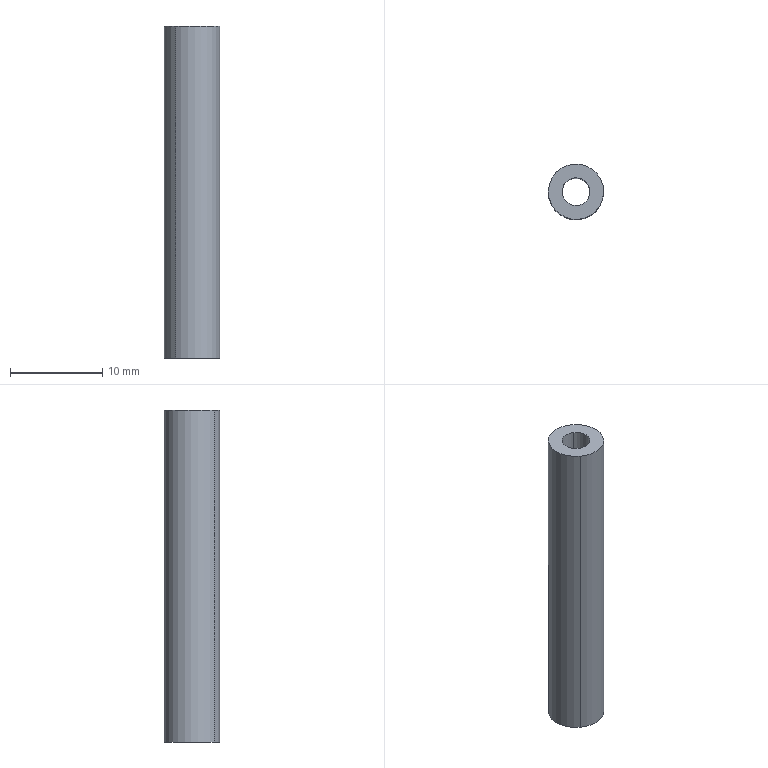Component | SolidWorks | UpperAndLowerPlateSupportColumn-3 | 1 solid | 6 faces | box 6 x 6 x 36 mm | volume 763 mm3 | cylinder 4 | plane 2 | commonest cylinder face diameters 3 x2 6 x2
build123d program:
from build123d import *

# Parameters (mm, degrees)
SKETCH1_R           = 3
SKETCH1_R_2         = 1.5
BOSS_EXTRUDE1_DEPTH = 36


with BuildPart() as part:
    # Sketch1 → Boss-Extrude1 (new body)
    with BuildSketch(Plane.XY):
        Circle(SKETCH1_R)
        Circle(SKETCH1_R_2, mode=Mode.SUBTRACT)
    extrude(amount=BOSS_EXTRUDE1_DEPTH)


solid = part.part

# Placed as in the assembly
solid = solid.moved(Location((14.261, -183.575, 1001.6), (0, 0, 0)))
STEP:
#1=CARTESIAN_POINT('',(0.5265,-7.275,40.85));
#2=VERTEX_POINT('',#1);
#3=CARTESIAN_POINT('',(0.5964,-7.18,40.85));
#4=VERTEX_POINT('',#3);
#5=CARTESIAN_POINT('',(0.5615,-7.227,40.85));
#6=DIRECTION('',(0.,0.,1.));
#7=DIRECTION('',(0.5916,0.8062,0.));
#8=AXIS2_PLACEMENT_3D('',#5,#6,#7);
#9=CIRCLE('',#8,0.05906);
#10=EDGE_CURVE('',#2,#4,#9,.T.);
#11=ORIENTED_EDGE('',*,*,#10,.T.);
#12=CARTESIAN_POINT('',(0.5964,-7.18,39.433));
#13=VERTEX_POINT('',#12);
#14=CARTESIAN_POINT('',(0.5964,-7.18,40.85));
#15=DIRECTION('',(0.,0.,-1.));
#16=VECTOR('',#15,39.37);
#17=LINE('',#14,#16);
#18=EDGE_CURVE('',#4,#13,#17,.T.);
#19=ORIENTED_EDGE('',*,*,#18,.T.);
#20=CARTESIAN_POINT('',(0.5265,-7.275,39.433));
#21=VERTEX_POINT('',#20);
#22=CARTESIAN_POINT('',(0.5615,-7.227,39.433));
#23=DIRECTION('',(0.,0.,1.));
#24=DIRECTION('',(0.5916,0.8062,0.));
#25=AXIS2_PLACEMENT_3D('',#22,#23,#24);
#26=CIRCLE('',#25,0.05906);
#27=EDGE_CURVE('',#21,#13,#26,.T.);
#28=ORIENTED_EDGE('',*,*,#27,.F.);
#29=CARTESIAN_POINT('',(0.5265,-7.275,40.85));
#30=DIRECTION('',(0.,0.,-1.));
#31=VECTOR('',#30,39.37);
#32=LINE('',#29,#31);
#33=EDGE_CURVE('',#2,#21,#32,.T.);
#34=ORIENTED_EDGE('',*,*,#33,.F.);
#35=EDGE_LOOP('',(#11,#19,#28,#34));
#36=FACE_OUTER_BOUND('',#35,.T.);
#37=CARTESIAN_POINT('',(0.5615,-7.227,40.85));
#38=DIRECTION('',(0.,0.,-1.));
#39=DIRECTION('',(-0.5916,-0.8062,0.));
#40=AXIS2_PLACEMENT_3D('',#37,#38,#39);
#41=CYLINDRICAL_SURFACE('',#40,0.05906);
#42=ADVANCED_FACE('',(#36),#41,.F.);
#43=CARTESIAN_POINT('',(0.6313,-7.132,40.85));
#44=VERTEX_POINT('',#43);
#45=CARTESIAN_POINT('',(0.4916,-7.323,40.85));
#46=VERTEX_POINT('',#45);
#47=CARTESIAN_POINT('',(0.5615,-7.227,40.85));
#48=DIRECTION('',(0.,0.,1.));
#49=DIRECTION('',(0.5916,0.8062,0.));
#50=AXIS2_PLACEMENT_3D('',#47,#48,#49);
#51=CIRCLE('',#50,0.1181);
#52=EDGE_CURVE('',#44,#46,#51,.T.);
#53=ORIENTED_EDGE('',*,*,#52,.F.);
#54=CARTESIAN_POINT('',(0.6313,-7.132,39.433));
#55=VERTEX_POINT('',#54);
#56=CARTESIAN_POINT('',(0.6313,-7.132,40.85));
#57=DIRECTION('',(0.,0.,-1.));
#58=VECTOR('',#57,39.37);
#59=LINE('',#56,#58);
#60=EDGE_CURVE('',#44,#55,#59,.T.);
#61=ORIENTED_EDGE('',*,*,#60,.T.);
#62=CARTESIAN_POINT('',(0.4916,-7.323,39.433));
#63=VERTEX_POINT('',#62);
#64=CARTESIAN_POINT('',(0.5615,-7.227,39.433));
#65=DIRECTION('',(0.,0.,1.));
#66=DIRECTION('',(0.5916,0.8062,0.));
#67=AXIS2_PLACEMENT_3D('',#64,#65,#66);
#68=CIRCLE('',#67,0.1181);
#69=EDGE_CURVE('',#55,#63,#68,.T.);
#70=ORIENTED_EDGE('',*,*,#69,.T.);
#71=CARTESIAN_POINT('',(0.4916,-7.323,40.85));
#72=DIRECTION('',(0.,0.,-1.));
#73=VECTOR('',#72,39.37);
#74=LINE('',#71,#73);
#75=EDGE_CURVE('',#46,#63,#74,.T.);
#76=ORIENTED_EDGE('',*,*,#75,.F.);
#77=EDGE_LOOP('',(#53,#61,#70,#76));
#78=FACE_OUTER_BOUND('',#77,.T.);
#79=CARTESIAN_POINT('',(0.5615,-7.227,40.85));
#80=DIRECTION('',(0.,0.,-1.));
#81=DIRECTION('',(-0.5916,-0.8062,0.));
#82=AXIS2_PLACEMENT_3D('',#79,#80,#81);
#83=CYLINDRICAL_SURFACE('',#82,0.1181);
#84=ADVANCED_FACE('',(#78),#83,.T.);
#85=CARTESIAN_POINT('',(0.5615,-7.227,40.85));
#86=DIRECTION('',(0.,0.,1.));
#87=DIRECTION('',(0.5916,0.8062,0.));
#88=AXIS2_PLACEMENT_3D('',#85,#86,#87);
#89=CIRCLE('',#88,0.1181);
#90=EDGE_CURVE('',#46,#44,#89,.T.);
#91=ORIENTED_EDGE('',*,*,#90,.T.);
#92=ORIENTED_EDGE('',*,*,#52,.T.);
#93=EDGE_LOOP('',(#91,#92));
#94=FACE_OUTER_BOUND('',#93,.T.);
#95=ORIENTED_EDGE('',*,*,#10,.F.);
#96=CARTESIAN_POINT('',(0.5615,-7.227,40.85));
#97=DIRECTION('',(0.,0.,1.));
#98=DIRECTION('',(0.5916,0.8062,0.));
#99=AXIS2_PLACEMENT_3D('',#96,#97,#98);
#100=CIRCLE('',#99,0.05906);
#101=EDGE_CURVE('',#4,#2,#100,.T.);
#102=ORIENTED_EDGE('',*,*,#101,.F.);
#103=EDGE_LOOP('',(#95,#102));
#104=FACE_BOUND('',#103,.T.);
#105=CARTESIAN_POINT('',(0.5615,-7.227,40.85));
#106=DIRECTION('',(0.,0.,1.));
#107=DIRECTION('',(0.5916,0.8062,0.));
#108=AXIS2_PLACEMENT_3D('',#105,#106,#107);
#109=PLANE('',#108);
#110=ADVANCED_FACE('',(#94,#104),#109,.T.);
#111=CARTESIAN_POINT('',(0.5615,-7.227,39.433));
#112=DIRECTION('',(0.,0.,1.));
#113=DIRECTION('',(0.5916,0.8062,0.));
#114=AXIS2_PLACEMENT_3D('',#111,#112,#113);
#115=CIRCLE('',#114,0.1181);
#116=EDGE_CURVE('',#63,#55,#115,.T.);
#117=ORIENTED_EDGE('',*,*,#116,.F.);
#118=ORIENTED_EDGE('',*,*,#69,.F.);
#119=EDGE_LOOP('',(#117,#118));
#120=FACE_OUTER_BOUND('',#119,.T.);
#121=ORIENTED_EDGE('',*,*,#27,.T.);
#122=CARTESIAN_POINT('',(0.5615,-7.227,39.433));
#123=DIRECTION('',(0.,0.,1.));
#124=DIRECTION('',(0.5916,0.8062,0.));
#125=AXIS2_PLACEMENT_3D('',#122,#123,#124);
#126=CIRCLE('',#125,0.05906);
#127=EDGE_CURVE('',#13,#21,#126,.T.);
#128=ORIENTED_EDGE('',*,*,#127,.T.);
#129=EDGE_LOOP('',(#121,#128));
#130=FACE_BOUND('',#129,.T.);
#131=CARTESIAN_POINT('',(0.5615,-7.227,39.433));
#132=DIRECTION('',(0.,0.,1.));
#133=DIRECTION('',(0.5916,0.8062,0.));
#134=AXIS2_PLACEMENT_3D('',#131,#132,#133);
#135=PLANE('',#134);
#136=ADVANCED_FACE('',(#120,#130),#135,.F.);
#137=ORIENTED_EDGE('',*,*,#60,.F.);
#138=ORIENTED_EDGE('',*,*,#90,.F.);
#139=ORIENTED_EDGE('',*,*,#75,.T.);
#140=ORIENTED_EDGE('',*,*,#116,.T.);
#141=EDGE_LOOP('',(#137,#138,#139,#140));
#142=FACE_OUTER_BOUND('',#141,.T.);
#143=CARTESIAN_POINT('',(0.5615,-7.227,40.85));
#144=DIRECTION('',(0.,0.,-1.));
#145=DIRECTION('',(-0.5916,-0.8062,0.));
#146=AXIS2_PLACEMENT_3D('',#143,#144,#145);
#147=CYLINDRICAL_SURFACE('',#146,0.1181);
#148=ADVANCED_FACE('',(#142),#147,.T.);
#149=ORIENTED_EDGE('',*,*,#18,.F.);
#150=ORIENTED_EDGE('',*,*,#101,.T.);
#151=ORIENTED_EDGE('',*,*,#33,.T.);
#152=ORIENTED_EDGE('',*,*,#127,.F.);
#153=EDGE_LOOP('',(#149,#150,#151,#152));
#154=FACE_OUTER_BOUND('',#153,.T.);
#155=CARTESIAN_POINT('',(0.5615,-7.227,40.85));
#156=DIRECTION('',(0.,0.,-1.));
#157=DIRECTION('',(-0.5916,-0.8062,0.));
#158=AXIS2_PLACEMENT_3D('',#155,#156,#157);
#159=CYLINDRICAL_SURFACE('',#158,0.05906);
#160=ADVANCED_FACE('',(#154),#159,.F.);
#161=CLOSED_SHELL('',(#42,#84,#110,#136,#148,#160));
#162=MANIFOLD_SOLID_BREP('',#161);
#163=CARTESIAN_POINT('',(0.,0.,0.));
#164=DIRECTION('',(0.,0.,1.));
#165=DIRECTION('',(1.,0.,0.));
#166=AXIS2_PLACEMENT_3D('',#163,#164,#165);
#167=(LENGTH_UNIT()NAMED_UNIT(*)SI_UNIT($,.METRE.));
#168=LENGTH_MEASURE_WITH_UNIT(LENGTH_MEASURE(0.0254),#167);
#169=DIMENSIONAL_EXPONENTS(1.,0.,0.,0.,0.,0.,0.);
#170=(CONVERSION_BASED_UNIT('',#168)LENGTH_UNIT()NAMED_UNIT(#169));
#171=UNCERTAINTY_MEASURE_WITH_UNIT(LENGTH_MEASURE(0.00001),#170,'','');
#172=(NAMED_UNIT(*)PLANE_ANGLE_UNIT()SI_UNIT($,.RADIAN.));
#173=(NAMED_UNIT(*)SI_UNIT($,.STERADIAN.)SOLID_ANGLE_UNIT());
#174=(GEOMETRIC_REPRESENTATION_CONTEXT(3)GLOBAL_UNCERTAINTY_ASSIGNED_CONTEXT((#171))GLOBAL_UNIT_ASSIGNED_CONTEXT((#170,#172,#173))REPRESENTATION_CONTEXT('',''));
#175=ADVANCED_BREP_SHAPE_REPRESENTATION('',(#162,#166),#174);
#176=COLOUR_RGB('',0.7922,0.8196,0.9333);
#177=FILL_AREA_STYLE_COLOUR('',#176);
#178=FILL_AREA_STYLE('',(#177));
#179=SURFACE_STYLE_FILL_AREA(#178);
#180=SURFACE_SIDE_STYLE('',(#179));
#181=SURFACE_STYLE_USAGE(.BOTH.,#180);
#182=PRESENTATION_STYLE_ASSIGNMENT((#181));
#183=STYLED_ITEM('',(#182),#162);
#184=PRESENTATION_LAYER_ASSIGNMENT('','',(#183));
#185=(LENGTH_UNIT()NAMED_UNIT(*)SI_UNIT($,.METRE.));
#186=LENGTH_MEASURE_WITH_UNIT(LENGTH_MEASURE(0.0254),#185);
#187=DIMENSIONAL_EXPONENTS(1.,0.,0.,0.,0.,0.,0.);
#188=(CONVERSION_BASED_UNIT('',#186)LENGTH_UNIT()NAMED_UNIT(#187));
#189=UNCERTAINTY_MEASURE_WITH_UNIT(LENGTH_MEASURE(0.00001),#188,'','');
#190=(NAMED_UNIT(*)PLANE_ANGLE_UNIT()SI_UNIT($,.RADIAN.));
#191=(NAMED_UNIT(*)SI_UNIT($,.STERADIAN.)SOLID_ANGLE_UNIT());
#192=(GEOMETRIC_REPRESENTATION_CONTEXT(3)GLOBAL_UNCERTAINTY_ASSIGNED_CONTEXT((#189))GLOBAL_UNIT_ASSIGNED_CONTEXT((#188,#190,#191))REPRESENTATION_CONTEXT('',''));
#193=MECHANICAL_DESIGN_GEOMETRIC_PRESENTATION_REPRESENTATION('',(#183),#192);